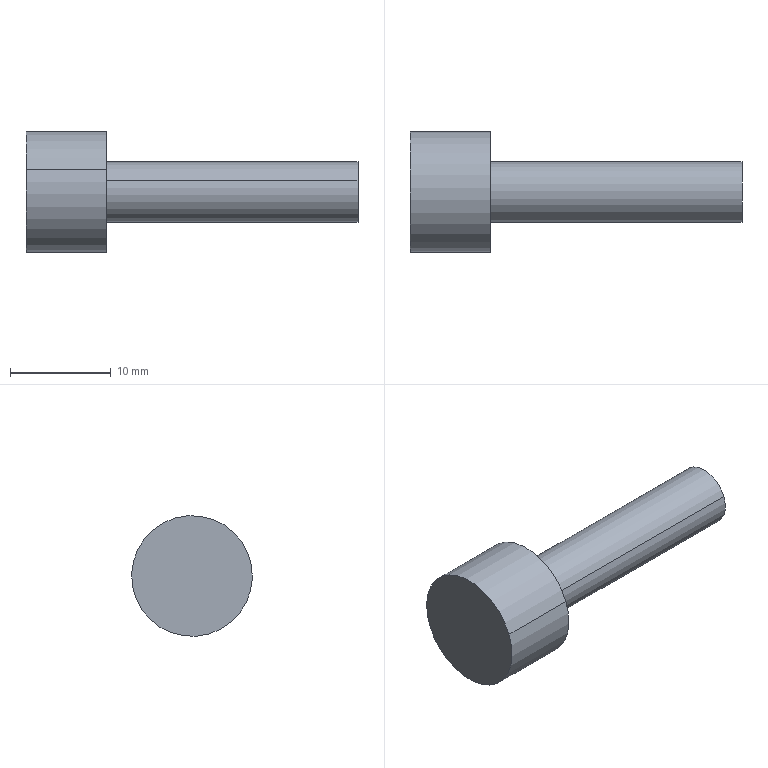Component | SolidWorks | 6-1 | 1 solid | 7 faces | box 33 x 12 x 12 mm | volume 1612 mm3 | cylinder 4 | plane 3 | commonest cylinder face diameters 6 x2 12 x2
build123d program:
from build123d import *

# Parameters (mm, degrees)
SKETCH1_R           = 6
BOSS_EXTRUDE1_DEPTH = 8
SKETCH2_R           = 3
BOSS_EXTRUDE2_DEPTH = 25


with BuildPart() as part:
    # Sketch1 → Boss-Extrude1 (new body)
    with BuildSketch(Plane.XY):
        Circle(SKETCH1_R)
    extrude(amount=BOSS_EXTRUDE1_DEPTH)

    # Sketch2 → Boss-Extrude2 (add)
    with BuildSketch(Plane.XY.offset(8)):
        Circle(SKETCH2_R)
    extrude(amount=BOSS_EXTRUDE2_DEPTH)


solid = part.part

# Placed as in the assembly
solid = solid.moved(Location((-205.043, 415.991, 747.751), (0, 90, 0)))
STEP:
#1=COLOUR_RGB('',0.7922,0.8196,0.9333);
#2=FILL_AREA_STYLE_COLOUR('',#1);
#3=FILL_AREA_STYLE('',(#2));
#4=SURFACE_STYLE_FILL_AREA(#3);
#5=SURFACE_SIDE_STYLE('',(#4));
#6=SURFACE_STYLE_USAGE(.BOTH.,#5);
#7=PRESENTATION_STYLE_ASSIGNMENT((#6));
#8=CARTESIAN_POINT('',(-6.773,16.268,29.483));
#9=VERTEX_POINT('',#8);
#10=CARTESIAN_POINT('',(-6.773,16.487,29.395));
#11=VERTEX_POINT('',#10);
#12=CARTESIAN_POINT('',(-6.773,16.378,29.439));
#13=DIRECTION('',(1.,0.,-0.));
#14=DIRECTION('',(0.,-0.9277,0.3734));
#15=AXIS2_PLACEMENT_3D('',#12,#13,#14);
#16=CIRCLE('',#15,0.1181);
#17=EDGE_CURVE('',#9,#11,#16,.T.);
#18=ORIENTED_EDGE('',*,*,#17,.F.);
#19=CARTESIAN_POINT('',(-7.758,16.268,29.483));
#20=VERTEX_POINT('',#19);
#21=CARTESIAN_POINT('',(-6.773,16.268,29.483));
#22=DIRECTION('',(-1.,-0.,0.));
#23=VECTOR('',#22,39.37);
#24=LINE('',#21,#23);
#25=EDGE_CURVE('',#9,#20,#24,.T.);
#26=ORIENTED_EDGE('',*,*,#25,.T.);
#27=CARTESIAN_POINT('',(-7.758,16.487,29.395));
#28=VERTEX_POINT('',#27);
#29=CARTESIAN_POINT('',(-7.758,16.378,29.439));
#30=DIRECTION('',(1.,0.,-0.));
#31=DIRECTION('',(0.,-0.9277,0.3734));
#32=AXIS2_PLACEMENT_3D('',#29,#30,#31);
#33=CIRCLE('',#32,0.1181);
#34=EDGE_CURVE('',#20,#28,#33,.T.);
#35=ORIENTED_EDGE('',*,*,#34,.T.);
#36=CARTESIAN_POINT('',(-6.773,16.487,29.395));
#37=DIRECTION('',(-1.,-0.,0.));
#38=VECTOR('',#37,39.37);
#39=LINE('',#36,#38);
#40=EDGE_CURVE('',#11,#28,#39,.T.);
#41=ORIENTED_EDGE('',*,*,#40,.F.);
#42=EDGE_LOOP('',(#18,#26,#35,#41));
#43=FACE_OUTER_BOUND('',#42,.T.);
#44=CARTESIAN_POINT('',(-6.773,16.378,29.439));
#45=DIRECTION('',(-1.,-0.,0.));
#46=DIRECTION('',(0.,0.9277,-0.3734));
#47=AXIS2_PLACEMENT_3D('',#44,#45,#46);
#48=CYLINDRICAL_SURFACE('',#47,0.1181);
#49=ADVANCED_FACE('',(#43),#48,.T.);
#50=CARTESIAN_POINT('',(-7.758,16.158,29.527));
#51=VERTEX_POINT('',#50);
#52=CARTESIAN_POINT('',(-7.758,16.597,29.351));
#53=VERTEX_POINT('',#52);
#54=CARTESIAN_POINT('',(-7.758,16.378,29.439));
#55=DIRECTION('',(1.,0.,-0.));
#56=DIRECTION('',(0.,-0.9277,0.3734));
#57=AXIS2_PLACEMENT_3D('',#54,#55,#56);
#58=CIRCLE('',#57,0.2362);
#59=EDGE_CURVE('',#51,#53,#58,.T.);
#60=ORIENTED_EDGE('',*,*,#59,.F.);
#61=CARTESIAN_POINT('',(-8.073,16.158,29.527));
#62=VERTEX_POINT('',#61);
#63=CARTESIAN_POINT('',(-7.758,16.158,29.527));
#64=DIRECTION('',(-1.,-0.,0.));
#65=VECTOR('',#64,39.37);
#66=LINE('',#63,#65);
#67=EDGE_CURVE('',#51,#62,#66,.T.);
#68=ORIENTED_EDGE('',*,*,#67,.T.);
#69=CARTESIAN_POINT('',(-8.073,16.597,29.351));
#70=VERTEX_POINT('',#69);
#71=CARTESIAN_POINT('',(-8.073,16.378,29.439));
#72=DIRECTION('',(1.,0.,-0.));
#73=DIRECTION('',(0.,-0.9277,0.3734));
#74=AXIS2_PLACEMENT_3D('',#71,#72,#73);
#75=CIRCLE('',#74,0.2362);
#76=EDGE_CURVE('',#62,#70,#75,.T.);
#77=ORIENTED_EDGE('',*,*,#76,.T.);
#78=CARTESIAN_POINT('',(-7.758,16.597,29.351));
#79=DIRECTION('',(-1.,-0.,0.));
#80=VECTOR('',#79,39.37);
#81=LINE('',#78,#80);
#82=EDGE_CURVE('',#53,#70,#81,.T.);
#83=ORIENTED_EDGE('',*,*,#82,.F.);
#84=EDGE_LOOP('',(#60,#68,#77,#83));
#85=FACE_OUTER_BOUND('',#84,.T.);
#86=CARTESIAN_POINT('',(-7.758,16.378,29.439));
#87=DIRECTION('',(-1.,-0.,0.));
#88=DIRECTION('',(0.,0.9277,-0.3734));
#89=AXIS2_PLACEMENT_3D('',#86,#87,#88);
#90=CYLINDRICAL_SURFACE('',#89,0.2362);
#91=ADVANCED_FACE('',(#85),#90,.T.);
#92=ORIENTED_EDGE('',*,*,#67,.F.);
#93=CARTESIAN_POINT('',(-7.758,16.378,29.439));
#94=DIRECTION('',(1.,0.,-0.));
#95=DIRECTION('',(0.,-0.9277,0.3734));
#96=AXIS2_PLACEMENT_3D('',#93,#94,#95);
#97=CIRCLE('',#96,0.2362);
#98=EDGE_CURVE('',#53,#51,#97,.T.);
#99=ORIENTED_EDGE('',*,*,#98,.F.);
#100=ORIENTED_EDGE('',*,*,#82,.T.);
#101=CARTESIAN_POINT('',(-8.073,16.378,29.439));
#102=DIRECTION('',(1.,0.,-0.));
#103=DIRECTION('',(0.,-0.9277,0.3734));
#104=AXIS2_PLACEMENT_3D('',#101,#102,#103);
#105=CIRCLE('',#104,0.2362);
#106=EDGE_CURVE('',#70,#62,#105,.T.);
#107=ORIENTED_EDGE('',*,*,#106,.T.);
#108=EDGE_LOOP('',(#92,#99,#100,#107));
#109=FACE_OUTER_BOUND('',#108,.T.);
#110=CARTESIAN_POINT('',(-7.758,16.378,29.439));
#111=DIRECTION('',(-1.,-0.,0.));
#112=DIRECTION('',(0.,0.9277,-0.3734));
#113=AXIS2_PLACEMENT_3D('',#110,#111,#112);
#114=CYLINDRICAL_SURFACE('',#113,0.2362);
#115=ADVANCED_FACE('',(#109),#114,.T.);
#116=CARTESIAN_POINT('',(-7.758,16.378,29.439));
#117=DIRECTION('',(1.,0.,-0.));
#118=DIRECTION('',(0.,-0.9277,0.3734));
#119=AXIS2_PLACEMENT_3D('',#116,#117,#118);
#120=CIRCLE('',#119,0.1181);
#121=EDGE_CURVE('',#28,#20,#120,.T.);
#122=ORIENTED_EDGE('',*,*,#121,.F.);
#123=ORIENTED_EDGE('',*,*,#34,.F.);
#124=EDGE_LOOP('',(#122,#123));
#125=FACE_BOUND('',#124,.T.);
#126=ORIENTED_EDGE('',*,*,#98,.T.);
#127=ORIENTED_EDGE('',*,*,#59,.T.);
#128=EDGE_LOOP('',(#126,#127));
#129=FACE_OUTER_BOUND('',#128,.T.);
#130=CARTESIAN_POINT('',(-7.758,16.378,29.439));
#131=DIRECTION('',(1.,0.,-0.));
#132=DIRECTION('',(0.,-0.9277,0.3734));
#133=AXIS2_PLACEMENT_3D('',#130,#131,#132);
#134=PLANE('',#133);
#135=ADVANCED_FACE('',(#125,#129),#134,.T.);
#136=ORIENTED_EDGE('',*,*,#106,.F.);
#137=ORIENTED_EDGE('',*,*,#76,.F.);
#138=EDGE_LOOP('',(#136,#137));
#139=FACE_OUTER_BOUND('',#138,.T.);
#140=CARTESIAN_POINT('',(-8.073,16.378,29.439));
#141=DIRECTION('',(1.,0.,-0.));
#142=DIRECTION('',(0.,-0.9277,0.3734));
#143=AXIS2_PLACEMENT_3D('',#140,#141,#142);
#144=PLANE('',#143);
#145=ADVANCED_FACE('',(#139),#144,.F.);
#146=ORIENTED_EDGE('',*,*,#25,.F.);
#147=CARTESIAN_POINT('',(-6.773,16.378,29.439));
#148=DIRECTION('',(1.,0.,-0.));
#149=DIRECTION('',(0.,-0.9277,0.3734));
#150=AXIS2_PLACEMENT_3D('',#147,#148,#149);
#151=CIRCLE('',#150,0.1181);
#152=EDGE_CURVE('',#11,#9,#151,.T.);
#153=ORIENTED_EDGE('',*,*,#152,.F.);
#154=ORIENTED_EDGE('',*,*,#40,.T.);
#155=ORIENTED_EDGE('',*,*,#121,.T.);
#156=EDGE_LOOP('',(#146,#153,#154,#155));
#157=FACE_OUTER_BOUND('',#156,.T.);
#158=CARTESIAN_POINT('',(-6.773,16.378,29.439));
#159=DIRECTION('',(-1.,-0.,0.));
#160=DIRECTION('',(0.,0.9277,-0.3734));
#161=AXIS2_PLACEMENT_3D('',#158,#159,#160);
#162=CYLINDRICAL_SURFACE('',#161,0.1181);
#163=ADVANCED_FACE('',(#157),#162,.T.);
#164=ORIENTED_EDGE('',*,*,#152,.T.);
#165=ORIENTED_EDGE('',*,*,#17,.T.);
#166=EDGE_LOOP('',(#164,#165));
#167=FACE_OUTER_BOUND('',#166,.T.);
#168=CARTESIAN_POINT('',(-6.773,16.378,29.439));
#169=DIRECTION('',(1.,0.,-0.));
#170=DIRECTION('',(0.,-0.9277,0.3734));
#171=AXIS2_PLACEMENT_3D('',#168,#169,#170);
#172=PLANE('',#171);
#173=ADVANCED_FACE('',(#167),#172,.T.);
#174=CLOSED_SHELL('',(#49,#91,#115,#135,#145,#163,#173));
#175=MANIFOLD_SOLID_BREP('',#174);
#176=STYLED_ITEM('',(#7),#175);
#177=PRESENTATION_LAYER_ASSIGNMENT('','',(#176));
#178=CARTESIAN_POINT('',(0.,0.,0.));
#179=DIRECTION('',(0.,0.,1.));
#180=DIRECTION('',(1.,0.,0.));
#181=AXIS2_PLACEMENT_3D('',#178,#179,#180);
#182=(LENGTH_UNIT()NAMED_UNIT(*)SI_UNIT($,.METRE.));
#183=LENGTH_MEASURE_WITH_UNIT(LENGTH_MEASURE(0.0254),#182);
#184=DIMENSIONAL_EXPONENTS(1.,0.,0.,0.,0.,0.,0.);
#185=(CONVERSION_BASED_UNIT('',#183)LENGTH_UNIT()NAMED_UNIT(#184));
#186=UNCERTAINTY_MEASURE_WITH_UNIT(LENGTH_MEASURE(0.00001),#185,'','');
#187=(NAMED_UNIT(*)PLANE_ANGLE_UNIT()SI_UNIT($,.RADIAN.));
#188=(NAMED_UNIT(*)SI_UNIT($,.STERADIAN.)SOLID_ANGLE_UNIT());
#189=(GEOMETRIC_REPRESENTATION_CONTEXT(3)GLOBAL_UNCERTAINTY_ASSIGNED_CONTEXT((#186))GLOBAL_UNIT_ASSIGNED_CONTEXT((#185,#187,#188))REPRESENTATION_CONTEXT('',''));
#190=ADVANCED_BREP_SHAPE_REPRESENTATION('',(#175,#181),#189);
#191=(LENGTH_UNIT()NAMED_UNIT(*)SI_UNIT($,.METRE.));
#192=LENGTH_MEASURE_WITH_UNIT(LENGTH_MEASURE(0.0254),#191);
#193=DIMENSIONAL_EXPONENTS(1.,0.,0.,0.,0.,0.,0.);
#194=(CONVERSION_BASED_UNIT('',#192)LENGTH_UNIT()NAMED_UNIT(#193));
#195=UNCERTAINTY_MEASURE_WITH_UNIT(LENGTH_MEASURE(0.00001),#194,'','');
#196=(NAMED_UNIT(*)PLANE_ANGLE_UNIT()SI_UNIT($,.RADIAN.));
#197=(NAMED_UNIT(*)SI_UNIT($,.STERADIAN.)SOLID_ANGLE_UNIT());
#198=(GEOMETRIC_REPRESENTATION_CONTEXT(3)GLOBAL_UNCERTAINTY_ASSIGNED_CONTEXT((#195))GLOBAL_UNIT_ASSIGNED_CONTEXT((#194,#196,#197))REPRESENTATION_CONTEXT('',''));
#199=MECHANICAL_DESIGN_GEOMETRIC_PRESENTATION_REPRESENTATION('',(#176),#198);